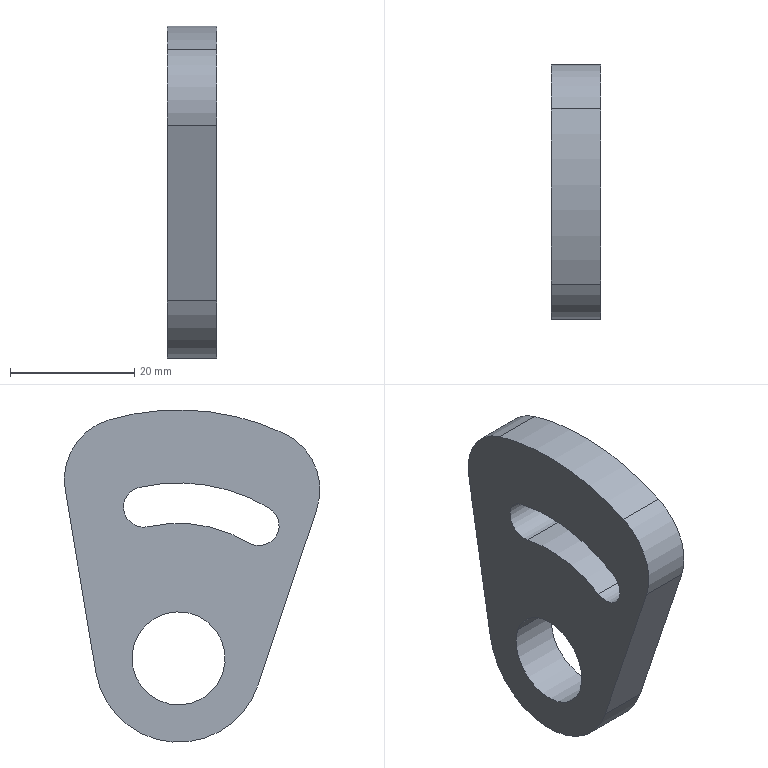Component | SolidWorks | MoldStopBlock001-1 | 1 solid | 15 faces | box 8 x 41.14 x 53.5 mm | volume 10642 mm3 | cylinder 11 | plane 4 | commonest cylinder face diameters 6.5 x3 15 x2 20 x2 27 x1 80 x1 56.5 x1 43.5 x1
build123d program:
from build123d import *

# Parameters (mm, degrees)
SKETCH1_R           = 7.5
BOSS_EXTRUDE1_DEPTH = 8
FILLET1_R           = 10


with BuildPart() as part:
    # Sketch1 → Boss-Extrude1 (new body)
    with BuildSketch(Plane.XY):
        with BuildLine():
            Line((-13.5, 0), (-13.5, -37.653))
            ThreePointArc((-13.5, -37.653), (9.677, -38.812), (29.597, -26.908))
            Line((29.597, -26.908), (11.92, 6.338))
            ThreePointArc((11.92, 6.338), (-3.266, 13.099), (-13.5, 0))
        make_face()
        Circle(SKETCH1_R, mode=Mode.SUBTRACT)
        with BuildLine():
            ThreePointArc((-6.215, -27.558), (4.597, -27.873), (14.735, -24.103))
            ThreePointArc((14.735, -24.103), (15.813, -19.635), (11.345, -18.557))
            ThreePointArc((11.345, -18.557), (3.539, -21.46), (-4.785, -21.217))
            ThreePointArc((-4.785, -21.217), (-8.67, -23.672), (-6.215, -27.558))
        make_face(mode=Mode.SUBTRACT)
    extrude(amount=BOSS_EXTRUDE1_DEPTH)

    # Fillet1
    fillet1_edges = [part.edges().sort_by_distance(p)[0] for p in [
        (29.597, -26.908, 4),
        (-13.5, -37.653, 4),
    ]]
    fillet(fillet1_edges, radius=FILLET1_R)


solid = part.part

# Placed as in the assembly
solid = solid.moved(Location((-256.896, -14.073, 553), (-71.548, -90, 0)))
STEP:
#1=COLOUR_RGB('',0.7922,0.8196,0.9333);
#2=FILL_AREA_STYLE_COLOUR('',#1);
#3=FILL_AREA_STYLE('',(#2));
#4=SURFACE_STYLE_FILL_AREA(#3);
#5=SURFACE_SIDE_STYLE('',(#4));
#6=SURFACE_STYLE_USAGE(.BOTH.,#5);
#7=PRESENTATION_STYLE_ASSIGNMENT((#6));
#8=CARTESIAN_POINT('',(-10.429,-0.9971,22.504));
#9=VERTEX_POINT('',#8);
#10=CARTESIAN_POINT('',(-10.429,-1.185,22.573));
#11=VERTEX_POINT('',#10);
#12=CARTESIAN_POINT('',(-10.429,-1.063,22.614));
#13=DIRECTION('',(-1.,0.,-0.));
#14=DIRECTION('',(0.,0.9486,0.3165));
#15=AXIS2_PLACEMENT_3D('',#12,#13,#14);
#16=CIRCLE('',#15,0.128);
#17=EDGE_CURVE('',#9,#11,#16,.T.);
#18=ORIENTED_EDGE('',*,*,#17,.T.);
#19=CARTESIAN_POINT('',(-10.114,-1.185,22.573));
#20=VERTEX_POINT('',#19);
#21=CARTESIAN_POINT('',(-10.429,-1.185,22.573));
#22=DIRECTION('',(1.,-0.,0.));
#23=VECTOR('',#22,39.37);
#24=LINE('',#21,#23);
#25=EDGE_CURVE('',#11,#20,#24,.T.);
#26=ORIENTED_EDGE('',*,*,#25,.T.);
#27=CARTESIAN_POINT('',(-10.114,-0.9971,22.504));
#28=VERTEX_POINT('',#27);
#29=CARTESIAN_POINT('',(-10.114,-1.063,22.614));
#30=DIRECTION('',(-1.,0.,-0.));
#31=DIRECTION('',(0.,0.9486,0.3165));
#32=AXIS2_PLACEMENT_3D('',#29,#30,#31);
#33=CIRCLE('',#32,0.128);
#34=EDGE_CURVE('',#28,#20,#33,.T.);
#35=ORIENTED_EDGE('',*,*,#34,.F.);
#36=CARTESIAN_POINT('',(-10.429,-0.9971,22.504));
#37=DIRECTION('',(1.,-0.,0.));
#38=VECTOR('',#37,39.37);
#39=LINE('',#36,#38);
#40=EDGE_CURVE('',#9,#28,#39,.T.);
#41=ORIENTED_EDGE('',*,*,#40,.F.);
#42=EDGE_LOOP('',(#18,#26,#35,#41));
#43=FACE_OUTER_BOUND('',#42,.T.);
#44=CARTESIAN_POINT('',(-10.429,-1.063,22.614));
#45=DIRECTION('',(1.,-0.,0.));
#46=DIRECTION('',(0.,-0.9486,-0.3165));
#47=AXIS2_PLACEMENT_3D('',#44,#45,#46);
#48=CYLINDRICAL_SURFACE('',#47,0.128);
#49=ADVANCED_FACE('',(#43),#48,.F.);
#50=CARTESIAN_POINT('',(-10.429,-0.8341,21.678));
#51=VERTEX_POINT('',#50);
#52=CARTESIAN_POINT('',(-10.429,-0.274,21.865));
#53=VERTEX_POINT('',#52);
#54=CARTESIAN_POINT('',(-10.429,-0.5541,21.772));
#55=DIRECTION('',(-1.,0.,-0.));
#56=DIRECTION('',(0.,0.9486,0.3165));
#57=AXIS2_PLACEMENT_3D('',#54,#55,#56);
#58=CIRCLE('',#57,0.2953);
#59=EDGE_CURVE('',#51,#53,#58,.T.);
#60=ORIENTED_EDGE('',*,*,#59,.T.);
#61=CARTESIAN_POINT('',(-10.114,-0.274,21.865));
#62=VERTEX_POINT('',#61);
#63=CARTESIAN_POINT('',(-10.429,-0.274,21.865));
#64=DIRECTION('',(1.,-0.,0.));
#65=VECTOR('',#64,39.37);
#66=LINE('',#63,#65);
#67=EDGE_CURVE('',#53,#62,#66,.T.);
#68=ORIENTED_EDGE('',*,*,#67,.T.);
#69=CARTESIAN_POINT('',(-10.114,-0.8341,21.678));
#70=VERTEX_POINT('',#69);
#71=CARTESIAN_POINT('',(-10.114,-0.5541,21.772));
#72=DIRECTION('',(-1.,0.,-0.));
#73=DIRECTION('',(0.,0.9486,0.3165));
#74=AXIS2_PLACEMENT_3D('',#71,#72,#73);
#75=CIRCLE('',#74,0.2953);
#76=EDGE_CURVE('',#70,#62,#75,.T.);
#77=ORIENTED_EDGE('',*,*,#76,.F.);
#78=CARTESIAN_POINT('',(-10.429,-0.8341,21.678));
#79=DIRECTION('',(1.,-0.,0.));
#80=VECTOR('',#79,39.37);
#81=LINE('',#78,#80);
#82=EDGE_CURVE('',#51,#70,#81,.T.);
#83=ORIENTED_EDGE('',*,*,#82,.F.);
#84=EDGE_LOOP('',(#60,#68,#77,#83));
#85=FACE_OUTER_BOUND('',#84,.T.);
#86=CARTESIAN_POINT('',(-10.429,-0.5541,21.772));
#87=DIRECTION('',(1.,-0.,0.));
#88=DIRECTION('',(0.,-0.9486,-0.3165));
#89=AXIS2_PLACEMENT_3D('',#86,#87,#88);
#90=CYLINDRICAL_SURFACE('',#89,0.2953);
#91=ADVANCED_FACE('',(#85),#90,.F.);
#92=CARTESIAN_POINT('',(-10.429,-1.058,21.603));
#93=VERTEX_POINT('',#92);
#94=CARTESIAN_POINT('',(-10.429,-1.429,22.716));
#95=VERTEX_POINT('',#94);
#96=CARTESIAN_POINT('',(-10.429,-1.058,21.603));
#97=DIRECTION('',(-0.,-0.3165,0.9486));
#98=VECTOR('',#97,39.37);
#99=LINE('',#96,#98);
#100=EDGE_CURVE('',#93,#95,#99,.T.);
#101=ORIENTED_EDGE('',*,*,#100,.T.);
#102=CARTESIAN_POINT('',(-10.429,-1.223,23.197));
#103=VERTEX_POINT('',#102);
#104=CARTESIAN_POINT('',(-10.429,-1.056,22.841));
#105=DIRECTION('',(-1.,0.,-0.));
#106=DIRECTION('',(0.,0.9486,0.3165));
#107=AXIS2_PLACEMENT_3D('',#104,#105,#106);
#108=CIRCLE('',#107,0.3937);
#109=EDGE_CURVE('',#95,#103,#108,.T.);
#110=ORIENTED_EDGE('',*,*,#109,.T.);
#111=CARTESIAN_POINT('',(-10.429,-0.1134,23.284));
#112=VERTEX_POINT('',#111);
#113=CARTESIAN_POINT('',(-10.429,-0.5541,21.772));
#114=DIRECTION('',(-1.,0.,-0.));
#115=DIRECTION('',(0.,0.9486,0.3165));
#116=AXIS2_PLACEMENT_3D('',#113,#114,#115);
#117=CIRCLE('',#116,1.575);
#118=EDGE_CURVE('',#103,#112,#117,.T.);
#119=ORIENTED_EDGE('',*,*,#118,.T.);
#120=CARTESIAN_POINT('',(-10.429,0.1647,22.84));
#121=VERTEX_POINT('',#120);
#122=CARTESIAN_POINT('',(-10.429,-0.2236,22.906));
#123=DIRECTION('',(-1.,0.,-0.));
#124=DIRECTION('',(0.,0.9486,0.3165));
#125=AXIS2_PLACEMENT_3D('',#122,#123,#124);
#126=CIRCLE('',#125,0.3937);
#127=EDGE_CURVE('',#112,#121,#126,.T.);
#128=ORIENTED_EDGE('',*,*,#127,.T.);
#129=CARTESIAN_POINT('',(-10.429,-0.02992,21.683));
#130=VERTEX_POINT('',#129);
#131=CARTESIAN_POINT('',(-10.429,-0.02992,21.683));
#132=DIRECTION('',(0.,-0.1659,-0.9861));
#133=VECTOR('',#132,39.37);
#134=LINE('',#131,#133);
#135=EDGE_CURVE('',#121,#130,#134,.T.);
#136=ORIENTED_EDGE('',*,*,#135,.T.);
#137=CARTESIAN_POINT('',(-10.429,-0.5541,21.772));
#138=DIRECTION('',(-1.,0.,-0.));
#139=DIRECTION('',(0.,0.9486,0.3165));
#140=AXIS2_PLACEMENT_3D('',#137,#138,#139);
#141=CIRCLE('',#140,0.5315);
#142=EDGE_CURVE('',#130,#93,#141,.T.);
#143=ORIENTED_EDGE('',*,*,#142,.T.);
#144=EDGE_LOOP('',(#101,#110,#119,#128,#136,#143));
#145=FACE_OUTER_BOUND('',#144,.T.);
#146=ORIENTED_EDGE('',*,*,#59,.F.);
#147=CARTESIAN_POINT('',(-10.429,-0.5541,21.772));
#148=DIRECTION('',(-1.,0.,-0.));
#149=DIRECTION('',(0.,0.9486,0.3165));
#150=AXIS2_PLACEMENT_3D('',#147,#148,#149);
#151=CIRCLE('',#150,0.2953);
#152=EDGE_CURVE('',#53,#51,#151,.T.);
#153=ORIENTED_EDGE('',*,*,#152,.F.);
#154=EDGE_LOOP('',(#146,#153));
#155=FACE_BOUND('',#154,.T.);
#156=CARTESIAN_POINT('',(-10.429,-1.13,22.723));
#157=VERTEX_POINT('',#156);
#158=CARTESIAN_POINT('',(-10.429,-0.3041,22.855));
#159=VERTEX_POINT('',#158);
#160=CARTESIAN_POINT('',(-10.429,-0.5541,21.772));
#161=DIRECTION('',(-1.,0.,-0.));
#162=DIRECTION('',(0.,0.9486,0.3165));
#163=AXIS2_PLACEMENT_3D('',#160,#161,#162);
#164=CIRCLE('',#163,1.112);
#165=EDGE_CURVE('',#157,#159,#164,.T.);
#166=ORIENTED_EDGE('',*,*,#165,.F.);
#167=CARTESIAN_POINT('',(-10.429,-1.063,22.614));
#168=DIRECTION('',(-1.,0.,-0.));
#169=DIRECTION('',(0.,0.9486,0.3165));
#170=AXIS2_PLACEMENT_3D('',#167,#168,#169);
#171=CIRCLE('',#170,0.128);
#172=EDGE_CURVE('',#11,#157,#171,.T.);
#173=ORIENTED_EDGE('',*,*,#172,.F.);
#174=ORIENTED_EDGE('',*,*,#17,.F.);
#175=CARTESIAN_POINT('',(-10.429,-0.3616,22.606));
#176=VERTEX_POINT('',#175);
#177=CARTESIAN_POINT('',(-10.429,-0.5541,21.772));
#178=DIRECTION('',(1.,-0.,0.));
#179=DIRECTION('',(0.,0.9486,0.3165));
#180=AXIS2_PLACEMENT_3D('',#177,#178,#179);
#181=CIRCLE('',#180,0.8563);
#182=EDGE_CURVE('',#176,#9,#181,.T.);
#183=ORIENTED_EDGE('',*,*,#182,.F.);
#184=CARTESIAN_POINT('',(-10.429,-0.3328,22.731));
#185=DIRECTION('',(-1.,0.,-0.));
#186=DIRECTION('',(0.,0.9486,0.3165));
#187=AXIS2_PLACEMENT_3D('',#184,#185,#186);
#188=CIRCLE('',#187,0.128);
#189=EDGE_CURVE('',#159,#176,#188,.T.);
#190=ORIENTED_EDGE('',*,*,#189,.F.);
#191=EDGE_LOOP('',(#166,#173,#174,#183,#190));
#192=FACE_BOUND('',#191,.T.);
#193=CARTESIAN_POINT('',(-10.429,-0.5541,21.772));
#194=DIRECTION('',(-1.,0.,-0.));
#195=DIRECTION('',(0.,0.9486,0.3165));
#196=AXIS2_PLACEMENT_3D('',#193,#194,#195);
#197=PLANE('',#196);
#198=ADVANCED_FACE('',(#145,#155,#192),#197,.T.);
#199=ORIENTED_EDGE('',*,*,#76,.T.);
#200=CARTESIAN_POINT('',(-10.114,-0.5541,21.772));
#201=DIRECTION('',(-1.,0.,-0.));
#202=DIRECTION('',(0.,0.9486,0.3165));
#203=AXIS2_PLACEMENT_3D('',#200,#201,#202);
#204=CIRCLE('',#203,0.2953);
#205=EDGE_CURVE('',#62,#70,#204,.T.);
#206=ORIENTED_EDGE('',*,*,#205,.T.);
#207=EDGE_LOOP('',(#199,#206));
#208=FACE_BOUND('',#207,.T.);
#209=CARTESIAN_POINT('',(-10.114,-1.223,23.197));
#210=VERTEX_POINT('',#209);
#211=CARTESIAN_POINT('',(-10.114,-0.1134,23.284));
#212=VERTEX_POINT('',#211);
#213=CARTESIAN_POINT('',(-10.114,-0.5541,21.772));
#214=DIRECTION('',(-1.,0.,-0.));
#215=DIRECTION('',(0.,0.9486,0.3165));
#216=AXIS2_PLACEMENT_3D('',#213,#214,#215);
#217=CIRCLE('',#216,1.575);
#218=EDGE_CURVE('',#210,#212,#217,.T.);
#219=ORIENTED_EDGE('',*,*,#218,.F.);
#220=CARTESIAN_POINT('',(-10.114,-1.429,22.716));
#221=VERTEX_POINT('',#220);
#222=CARTESIAN_POINT('',(-10.114,-1.056,22.841));
#223=DIRECTION('',(1.,-0.,0.));
#224=DIRECTION('',(0.,0.9486,0.3165));
#225=AXIS2_PLACEMENT_3D('',#222,#223,#224);
#226=CIRCLE('',#225,0.3937);
#227=EDGE_CURVE('',#210,#221,#226,.T.);
#228=ORIENTED_EDGE('',*,*,#227,.T.);
#229=CARTESIAN_POINT('',(-10.114,-1.058,21.603));
#230=VERTEX_POINT('',#229);
#231=CARTESIAN_POINT('',(-10.114,-1.058,21.603));
#232=DIRECTION('',(-0.,-0.3165,0.9486));
#233=VECTOR('',#232,39.37);
#234=LINE('',#231,#233);
#235=EDGE_CURVE('',#230,#221,#234,.T.);
#236=ORIENTED_EDGE('',*,*,#235,.F.);
#237=CARTESIAN_POINT('',(-10.114,-0.02992,21.683));
#238=VERTEX_POINT('',#237);
#239=CARTESIAN_POINT('',(-10.114,-0.5541,21.772));
#240=DIRECTION('',(-1.,0.,-0.));
#241=DIRECTION('',(0.,0.9486,0.3165));
#242=AXIS2_PLACEMENT_3D('',#239,#240,#241);
#243=CIRCLE('',#242,0.5315);
#244=EDGE_CURVE('',#238,#230,#243,.T.);
#245=ORIENTED_EDGE('',*,*,#244,.F.);
#246=CARTESIAN_POINT('',(-10.114,0.1647,22.84));
#247=VERTEX_POINT('',#246);
#248=CARTESIAN_POINT('',(-10.114,-0.02992,21.683));
#249=DIRECTION('',(0.,-0.1659,-0.9861));
#250=VECTOR('',#249,39.37);
#251=LINE('',#248,#250);
#252=EDGE_CURVE('',#247,#238,#251,.T.);
#253=ORIENTED_EDGE('',*,*,#252,.F.);
#254=CARTESIAN_POINT('',(-10.114,-0.2236,22.906));
#255=DIRECTION('',(1.,-0.,0.));
#256=DIRECTION('',(0.,0.9486,0.3165));
#257=AXIS2_PLACEMENT_3D('',#254,#255,#256);
#258=CIRCLE('',#257,0.3937);
#259=EDGE_CURVE('',#247,#212,#258,.T.);
#260=ORIENTED_EDGE('',*,*,#259,.T.);
#261=EDGE_LOOP('',(#219,#228,#236,#245,#253,#260));
#262=FACE_OUTER_BOUND('',#261,.T.);
#263=ORIENTED_EDGE('',*,*,#34,.T.);
#264=CARTESIAN_POINT('',(-10.114,-1.13,22.723));
#265=VERTEX_POINT('',#264);
#266=CARTESIAN_POINT('',(-10.114,-1.063,22.614));
#267=DIRECTION('',(-1.,0.,-0.));
#268=DIRECTION('',(0.,0.9486,0.3165));
#269=AXIS2_PLACEMENT_3D('',#266,#267,#268);
#270=CIRCLE('',#269,0.128);
#271=EDGE_CURVE('',#20,#265,#270,.T.);
#272=ORIENTED_EDGE('',*,*,#271,.T.);
#273=CARTESIAN_POINT('',(-10.114,-0.3041,22.855));
#274=VERTEX_POINT('',#273);
#275=CARTESIAN_POINT('',(-10.114,-0.5541,21.772));
#276=DIRECTION('',(-1.,0.,-0.));
#277=DIRECTION('',(0.,0.9486,0.3165));
#278=AXIS2_PLACEMENT_3D('',#275,#276,#277);
#279=CIRCLE('',#278,1.112);
#280=EDGE_CURVE('',#265,#274,#279,.T.);
#281=ORIENTED_EDGE('',*,*,#280,.T.);
#282=CARTESIAN_POINT('',(-10.114,-0.3616,22.606));
#283=VERTEX_POINT('',#282);
#284=CARTESIAN_POINT('',(-10.114,-0.3328,22.731));
#285=DIRECTION('',(-1.,0.,-0.));
#286=DIRECTION('',(0.,0.9486,0.3165));
#287=AXIS2_PLACEMENT_3D('',#284,#285,#286);
#288=CIRCLE('',#287,0.128);
#289=EDGE_CURVE('',#274,#283,#288,.T.);
#290=ORIENTED_EDGE('',*,*,#289,.T.);
#291=CARTESIAN_POINT('',(-10.114,-0.5541,21.772));
#292=DIRECTION('',(1.,-0.,0.));
#293=DIRECTION('',(0.,0.9486,0.3165));
#294=AXIS2_PLACEMENT_3D('',#291,#292,#293);
#295=CIRCLE('',#294,0.8563);
#296=EDGE_CURVE('',#283,#28,#295,.T.);
#297=ORIENTED_EDGE('',*,*,#296,.T.);
#298=EDGE_LOOP('',(#263,#272,#281,#290,#297));
#299=FACE_BOUND('',#298,.T.);
#300=CARTESIAN_POINT('',(-10.114,-0.5541,21.772));
#301=DIRECTION('',(-1.,0.,-0.));
#302=DIRECTION('',(0.,0.9486,0.3165));
#303=AXIS2_PLACEMENT_3D('',#300,#301,#302);
#304=PLANE('',#303);
#305=ADVANCED_FACE('',(#208,#262,#299),#304,.F.);
#306=ORIENTED_EDGE('',*,*,#244,.T.);
#307=CARTESIAN_POINT('',(-10.429,-1.058,21.603));
#308=DIRECTION('',(1.,-0.,0.));
#309=VECTOR('',#308,39.37);
#310=LINE('',#307,#309);
#311=EDGE_CURVE('',#93,#230,#310,.T.);
#312=ORIENTED_EDGE('',*,*,#311,.F.);
#313=ORIENTED_EDGE('',*,*,#142,.F.);
#314=CARTESIAN_POINT('',(-10.429,-0.02992,21.683));
#315=DIRECTION('',(1.,-0.,0.));
#316=VECTOR('',#315,39.37);
#317=LINE('',#314,#316);
#318=EDGE_CURVE('',#130,#238,#317,.T.);
#319=ORIENTED_EDGE('',*,*,#318,.T.);
#320=EDGE_LOOP('',(#306,#312,#313,#319));
#321=FACE_OUTER_BOUND('',#320,.T.);
#322=CARTESIAN_POINT('',(-10.429,-0.5541,21.772));
#323=DIRECTION('',(1.,-0.,0.));
#324=DIRECTION('',(0.,-0.9486,-0.3165));
#325=AXIS2_PLACEMENT_3D('',#322,#323,#324);
#326=CYLINDRICAL_SURFACE('',#325,0.5315);
#327=ADVANCED_FACE('',(#321),#326,.T.);
#328=ORIENTED_EDGE('',*,*,#235,.T.);
#329=CARTESIAN_POINT('',(-10.429,-1.429,22.716));
#330=DIRECTION('',(-1.,0.,-0.));
#331=VECTOR('',#330,39.37);
#332=LINE('',#329,#331);
#333=EDGE_CURVE('',#221,#95,#332,.T.);
#334=ORIENTED_EDGE('',*,*,#333,.T.);
#335=ORIENTED_EDGE('',*,*,#100,.F.);
#336=ORIENTED_EDGE('',*,*,#311,.T.);
#337=EDGE_LOOP('',(#328,#334,#335,#336));
#338=FACE_OUTER_BOUND('',#337,.T.);
#339=CARTESIAN_POINT('',(-10.429,-1.058,21.603));
#340=DIRECTION('',(0.,0.9486,0.3165));
#341=DIRECTION('',(0.,0.3165,-0.9486));
#342=AXIS2_PLACEMENT_3D('',#339,#340,#341);
#343=PLANE('',#342);
#344=ADVANCED_FACE('',(#338),#343,.F.);
#345=ORIENTED_EDGE('',*,*,#118,.F.);
#346=CARTESIAN_POINT('',(-10.429,-1.223,23.197));
#347=DIRECTION('',(1.,-0.,0.));
#348=VECTOR('',#347,39.37);
#349=LINE('',#346,#348);
#350=EDGE_CURVE('',#103,#210,#349,.T.);
#351=ORIENTED_EDGE('',*,*,#350,.T.);
#352=ORIENTED_EDGE('',*,*,#218,.T.);
#353=CARTESIAN_POINT('',(-10.429,-0.1134,23.284));
#354=DIRECTION('',(-1.,0.,-0.));
#355=VECTOR('',#354,39.37);
#356=LINE('',#353,#355);
#357=EDGE_CURVE('',#212,#112,#356,.T.);
#358=ORIENTED_EDGE('',*,*,#357,.T.);
#359=EDGE_LOOP('',(#345,#351,#352,#358));
#360=FACE_OUTER_BOUND('',#359,.T.);
#361=CARTESIAN_POINT('',(-10.429,-0.5541,21.772));
#362=DIRECTION('',(1.,-0.,0.));
#363=DIRECTION('',(0.,-0.9486,-0.3165));
#364=AXIS2_PLACEMENT_3D('',#361,#362,#363);
#365=CYLINDRICAL_SURFACE('',#364,1.575);
#366=ADVANCED_FACE('',(#360),#365,.T.);
#367=ORIENTED_EDGE('',*,*,#135,.F.);
#368=CARTESIAN_POINT('',(-10.429,0.1647,22.84));
#369=DIRECTION('',(1.,-0.,0.));
#370=VECTOR('',#369,39.37);
#371=LINE('',#368,#370);
#372=EDGE_CURVE('',#121,#247,#371,.T.);
#373=ORIENTED_EDGE('',*,*,#372,.T.);
#374=ORIENTED_EDGE('',*,*,#252,.T.);
#375=ORIENTED_EDGE('',*,*,#318,.F.);
#376=EDGE_LOOP('',(#367,#373,#374,#375));
#377=FACE_OUTER_BOUND('',#376,.T.);
#378=CARTESIAN_POINT('',(-10.429,-0.02992,21.683));
#379=DIRECTION('',(-0.,-0.9861,0.1659));
#380=DIRECTION('',(-0.,0.1659,0.9861));
#381=AXIS2_PLACEMENT_3D('',#378,#379,#380);
#382=PLANE('',#381);
#383=ADVANCED_FACE('',(#377),#382,.F.);
#384=ORIENTED_EDGE('',*,*,#67,.F.);
#385=ORIENTED_EDGE('',*,*,#152,.T.);
#386=ORIENTED_EDGE('',*,*,#82,.T.);
#387=ORIENTED_EDGE('',*,*,#205,.F.);
#388=EDGE_LOOP('',(#384,#385,#386,#387));
#389=FACE_OUTER_BOUND('',#388,.T.);
#390=CARTESIAN_POINT('',(-10.429,-0.5541,21.772));
#391=DIRECTION('',(1.,-0.,0.));
#392=DIRECTION('',(0.,-0.9486,-0.3165));
#393=AXIS2_PLACEMENT_3D('',#390,#391,#392);
#394=CYLINDRICAL_SURFACE('',#393,0.2953);
#395=ADVANCED_FACE('',(#389),#394,.F.);
#396=ORIENTED_EDGE('',*,*,#25,.F.);
#397=ORIENTED_EDGE('',*,*,#172,.T.);
#398=CARTESIAN_POINT('',(-10.429,-1.13,22.723));
#399=DIRECTION('',(1.,-0.,0.));
#400=VECTOR('',#399,39.37);
#401=LINE('',#398,#400);
#402=EDGE_CURVE('',#157,#265,#401,.T.);
#403=ORIENTED_EDGE('',*,*,#402,.T.);
#404=ORIENTED_EDGE('',*,*,#271,.F.);
#405=EDGE_LOOP('',(#396,#397,#403,#404));
#406=FACE_OUTER_BOUND('',#405,.T.);
#407=CARTESIAN_POINT('',(-10.429,-1.063,22.614));
#408=DIRECTION('',(1.,-0.,0.));
#409=DIRECTION('',(0.,-0.9486,-0.3165));
#410=AXIS2_PLACEMENT_3D('',#407,#408,#409);
#411=CYLINDRICAL_SURFACE('',#410,0.128);
#412=ADVANCED_FACE('',(#406),#411,.F.);
#413=ORIENTED_EDGE('',*,*,#280,.F.);
#414=ORIENTED_EDGE('',*,*,#402,.F.);
#415=ORIENTED_EDGE('',*,*,#165,.T.);
#416=CARTESIAN_POINT('',(-10.429,-0.3041,22.855));
#417=DIRECTION('',(1.,-0.,0.));
#418=VECTOR('',#417,39.37);
#419=LINE('',#416,#418);
#420=EDGE_CURVE('',#159,#274,#419,.T.);
#421=ORIENTED_EDGE('',*,*,#420,.T.);
#422=EDGE_LOOP('',(#413,#414,#415,#421));
#423=FACE_OUTER_BOUND('',#422,.T.);
#424=CARTESIAN_POINT('',(-10.429,-0.5541,21.772));
#425=DIRECTION('',(1.,-0.,0.));
#426=DIRECTION('',(0.,-0.9486,-0.3165));
#427=AXIS2_PLACEMENT_3D('',#424,#425,#426);
#428=CYLINDRICAL_SURFACE('',#427,1.112);
#429=ADVANCED_FACE('',(#423),#428,.F.);
#430=ORIENTED_EDGE('',*,*,#289,.F.);
#431=ORIENTED_EDGE('',*,*,#420,.F.);
#432=ORIENTED_EDGE('',*,*,#189,.T.);
#433=CARTESIAN_POINT('',(-10.429,-0.3616,22.606));
#434=DIRECTION('',(1.,-0.,0.));
#435=VECTOR('',#434,39.37);
#436=LINE('',#433,#435);
#437=EDGE_CURVE('',#176,#283,#436,.T.);
#438=ORIENTED_EDGE('',*,*,#437,.T.);
#439=EDGE_LOOP('',(#430,#431,#432,#438));
#440=FACE_OUTER_BOUND('',#439,.T.);
#441=CARTESIAN_POINT('',(-10.429,-0.3328,22.731));
#442=DIRECTION('',(1.,-0.,0.));
#443=DIRECTION('',(0.,-0.9486,-0.3165));
#444=AXIS2_PLACEMENT_3D('',#441,#442,#443);
#445=CYLINDRICAL_SURFACE('',#444,0.128);
#446=ADVANCED_FACE('',(#440),#445,.F.);
#447=ORIENTED_EDGE('',*,*,#296,.F.);
#448=ORIENTED_EDGE('',*,*,#437,.F.);
#449=ORIENTED_EDGE('',*,*,#182,.T.);
#450=ORIENTED_EDGE('',*,*,#40,.T.);
#451=EDGE_LOOP('',(#447,#448,#449,#450));
#452=FACE_OUTER_BOUND('',#451,.T.);
#453=CARTESIAN_POINT('',(-10.429,-0.5541,21.772));
#454=DIRECTION('',(1.,-0.,0.));
#455=DIRECTION('',(0.,-0.9486,-0.3165));
#456=AXIS2_PLACEMENT_3D('',#453,#454,#455);
#457=CYLINDRICAL_SURFACE('',#456,0.8563);
#458=ADVANCED_FACE('',(#452),#457,.T.);
#459=ORIENTED_EDGE('',*,*,#109,.F.);
#460=ORIENTED_EDGE('',*,*,#333,.F.);
#461=ORIENTED_EDGE('',*,*,#227,.F.);
#462=ORIENTED_EDGE('',*,*,#350,.F.);
#463=EDGE_LOOP('',(#459,#460,#461,#462));
#464=FACE_OUTER_BOUND('',#463,.T.);
#465=CARTESIAN_POINT('',(-10.429,-1.056,22.841));
#466=DIRECTION('',(1.,-0.,0.));
#467=DIRECTION('',(0.,-0.9486,-0.3165));
#468=AXIS2_PLACEMENT_3D('',#465,#466,#467);
#469=CYLINDRICAL_SURFACE('',#468,0.3937);
#470=ADVANCED_FACE('',(#464),#469,.T.);
#471=ORIENTED_EDGE('',*,*,#127,.F.);
#472=ORIENTED_EDGE('',*,*,#357,.F.);
#473=ORIENTED_EDGE('',*,*,#259,.F.);
#474=ORIENTED_EDGE('',*,*,#372,.F.);
#475=EDGE_LOOP('',(#471,#472,#473,#474));
#476=FACE_OUTER_BOUND('',#475,.T.);
#477=CARTESIAN_POINT('',(-10.429,-0.2236,22.906));
#478=DIRECTION('',(1.,-0.,0.));
#479=DIRECTION('',(0.,-0.9486,-0.3165));
#480=AXIS2_PLACEMENT_3D('',#477,#478,#479);
#481=CYLINDRICAL_SURFACE('',#480,0.3937);
#482=ADVANCED_FACE('',(#476),#481,.T.);
#483=CLOSED_SHELL('',(#49,#91,#198,#305,#327,#344,#366,#383,#395,#412,#429,#446,#458,#470,#482));
#484=MANIFOLD_SOLID_BREP('',#483);
#485=STYLED_ITEM('',(#7),#484);
#486=PRESENTATION_LAYER_ASSIGNMENT('','',(#485));
#487=CARTESIAN_POINT('',(0.,0.,0.));
#488=DIRECTION('',(0.,0.,1.));
#489=DIRECTION('',(1.,0.,0.));
#490=AXIS2_PLACEMENT_3D('',#487,#488,#489);
#491=(LENGTH_UNIT()NAMED_UNIT(*)SI_UNIT($,.METRE.));
#492=LENGTH_MEASURE_WITH_UNIT(LENGTH_MEASURE(0.0254),#491);
#493=DIMENSIONAL_EXPONENTS(1.,0.,0.,0.,0.,0.,0.);
#494=(CONVERSION_BASED_UNIT('',#492)LENGTH_UNIT()NAMED_UNIT(#493));
#495=UNCERTAINTY_MEASURE_WITH_UNIT(LENGTH_MEASURE(0.00001),#494,'','');
#496=(NAMED_UNIT(*)PLANE_ANGLE_UNIT()SI_UNIT($,.RADIAN.));
#497=(NAMED_UNIT(*)SI_UNIT($,.STERADIAN.)SOLID_ANGLE_UNIT());
#498=(GEOMETRIC_REPRESENTATION_CONTEXT(3)GLOBAL_UNCERTAINTY_ASSIGNED_CONTEXT((#495))GLOBAL_UNIT_ASSIGNED_CONTEXT((#494,#496,#497))REPRESENTATION_CONTEXT('',''));
#499=ADVANCED_BREP_SHAPE_REPRESENTATION('',(#484,#490),#498);
#500=(LENGTH_UNIT()NAMED_UNIT(*)SI_UNIT($,.METRE.));
#501=LENGTH_MEASURE_WITH_UNIT(LENGTH_MEASURE(0.0254),#500);
#502=DIMENSIONAL_EXPONENTS(1.,0.,0.,0.,0.,0.,0.);
#503=(CONVERSION_BASED_UNIT('',#501)LENGTH_UNIT()NAMED_UNIT(#502));
#504=UNCERTAINTY_MEASURE_WITH_UNIT(LENGTH_MEASURE(0.00001),#503,'','');
#505=(NAMED_UNIT(*)PLANE_ANGLE_UNIT()SI_UNIT($,.RADIAN.));
#506=(NAMED_UNIT(*)SI_UNIT($,.STERADIAN.)SOLID_ANGLE_UNIT());
#507=(GEOMETRIC_REPRESENTATION_CONTEXT(3)GLOBAL_UNCERTAINTY_ASSIGNED_CONTEXT((#504))GLOBAL_UNIT_ASSIGNED_CONTEXT((#503,#505,#506))REPRESENTATION_CONTEXT('',''));
#508=MECHANICAL_DESIGN_GEOMETRIC_PRESENTATION_REPRESENTATION('',(#485),#507);